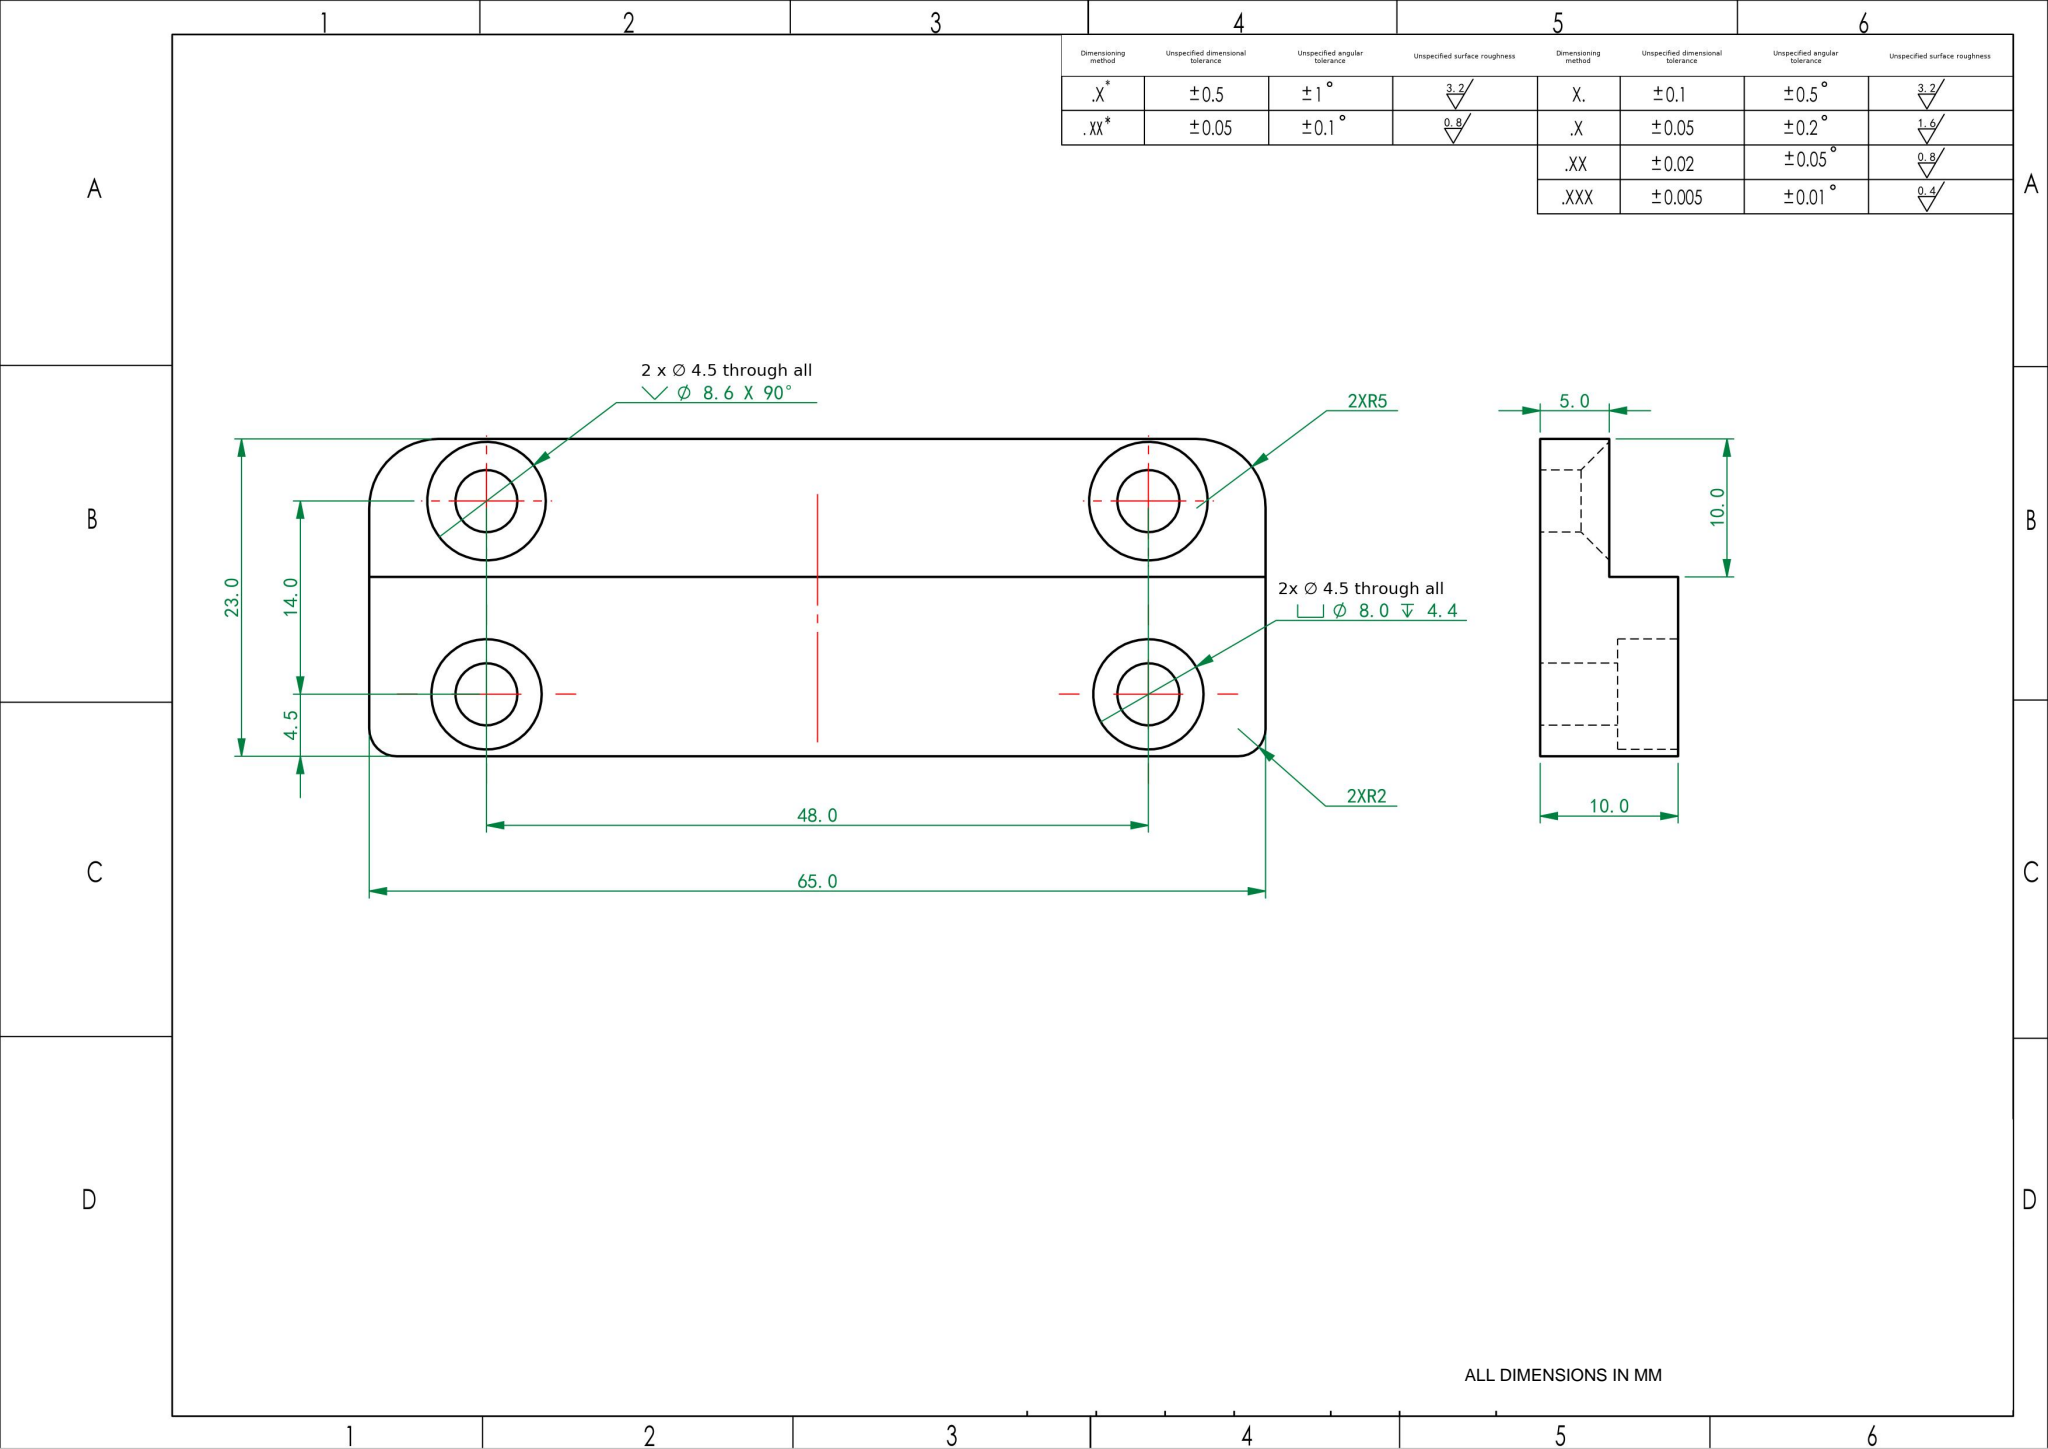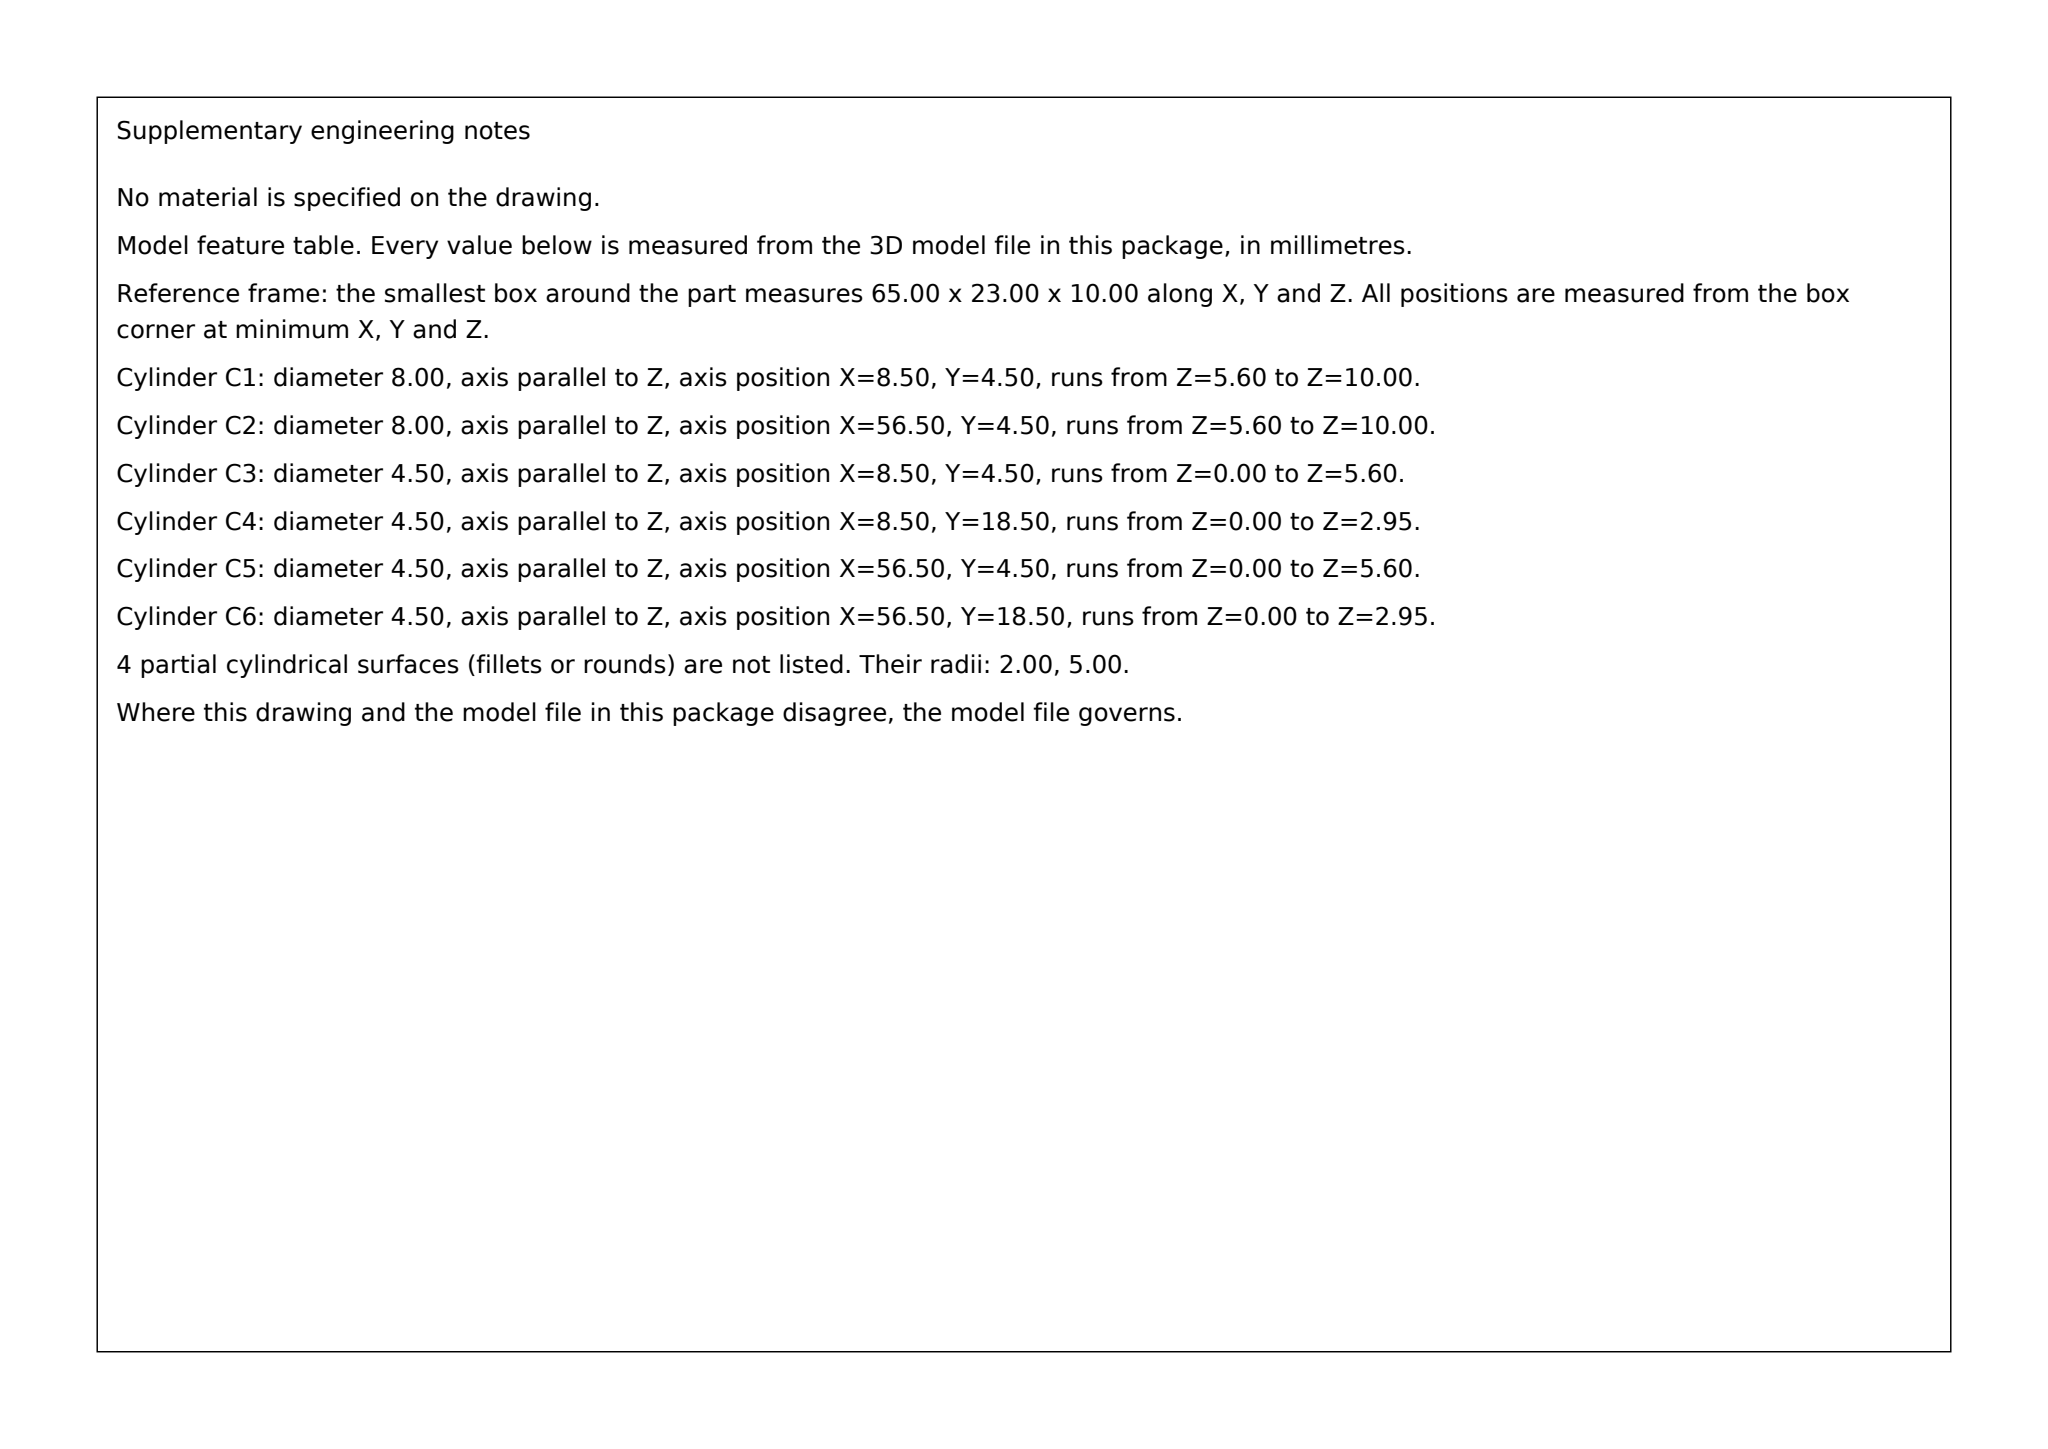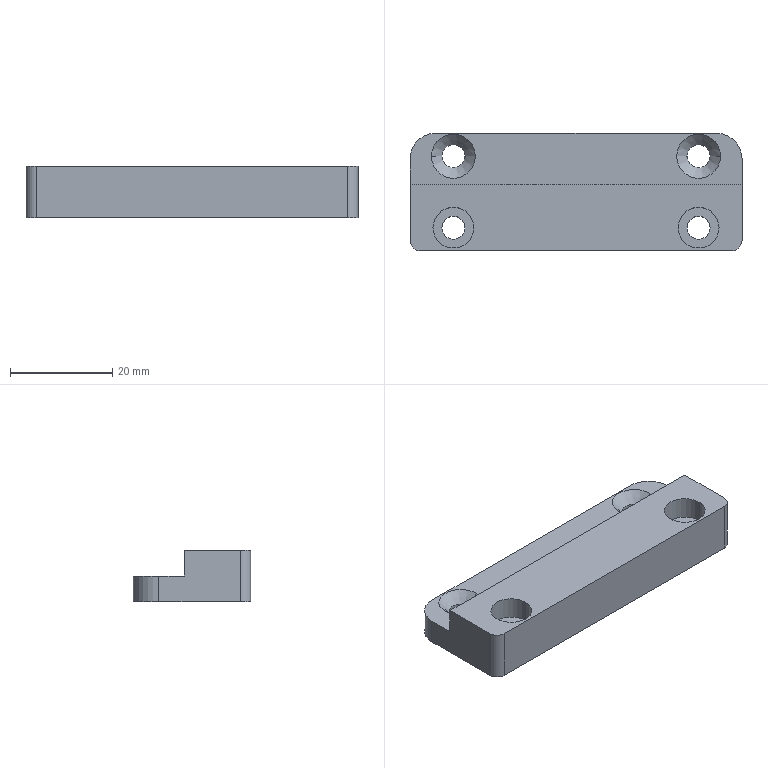Part | SolidWorks | mm | 1 solid | 30 faces | box 65 x 23 x 10 mm | volume 10772 mm3 | cylinder 16 | plane 10 | cone 4 | commonest cylinder face diameters 4.5 x8 8 x4 10 x2 4 x2
build123d program:
from build123d import *

# Parameters (mm, degrees)
SKETCH1_W                                         = 65
SKETCH1_H                                         = 23
BOSS_EXTRUDE1_DEPTH                               = 10
M4_HEX_SOCKET_HEAD_CAP_SCREW_CBORE2_D             = 4.5
M4_HEX_SOCKET_HEAD_CAP_SCREW_CBORE2_CBORE_D       = 8
M4_HEX_SOCKET_HEAD_CAP_SCREW_CBORE2_CBORE_DEPTH   = 4.4
SKETCH4_W                                         = 65
SKETCH4_H                                         = 10
CUT_EXTRUDE1_DEPTH                                = 5
FILLET1_R                                         = 5
FILLET2_R                                         = 2
HOLE_SIZE_ACCORDING_TO_PHILLIPS_COUNT_D           = 4.5
HOLE_SIZE_ACCORDING_TO_PHILLIPS_COUNT_CSINK_D     = 8.6
HOLE_SIZE_ACCORDING_TO_PHILLIPS_COUNT_CSINK_ANGLE = 90


with BuildPart() as part:
    # Sketch1 → Boss-Extrude1 (new body)
    with BuildSketch(Plane.XY):
        Rectangle(SKETCH1_W, SKETCH1_H)
    extrude(amount=BOSS_EXTRUDE1_DEPTH)

    # M4 Hex Socket Head Cap Screw CBORE2 (through all)
    with Locations(Plane(origin=(-24, 7, 10), x_dir=(1, 0, 0), z_dir=(0, 0, 1))):
        with Locations((0, 0), (0, -14), (48, -14), (48, 0)):
            CounterBoreHole(M4_HEX_SOCKET_HEAD_CAP_SCREW_CBORE2_D / 2, M4_HEX_SOCKET_HEAD_CAP_SCREW_CBORE2_CBORE_D / 2, M4_HEX_SOCKET_HEAD_CAP_SCREW_CBORE2_CBORE_DEPTH)

    # Sketch4 → Cut-Extrude1 (cut)
    with BuildSketch(Plane.XY.offset(10)):
        with Locations((0, 6.5)):
            Rectangle(SKETCH4_W, SKETCH4_H)
    extrude(amount=-CUT_EXTRUDE1_DEPTH, mode=Mode.SUBTRACT)

    # Fillet1
    fillet1_edges = [part.edges().sort_by_distance(p)[0] for p in [
        (-32.5, 11.5, 2.5),
        (32.5, 11.5, 2.5),
    ]]
    fillet(fillet1_edges, radius=FILLET1_R)

    # Fillet2
    fillet2_edges = [part.edges().sort_by_distance(p)[0] for p in [
        (32.5, -11.5, 5),
        (-32.5, -11.5, 5),
    ]]
    fillet(fillet2_edges, radius=FILLET2_R)

    # Hole Size _ according to Phillips_ Count (through all)
    with Locations(Plane(origin=(-24, 7, 5), x_dir=(1, 0, 0), z_dir=(0, 0, 1))):
        with Locations((0, 0), (48, 0)):
            CounterSinkHole(HOLE_SIZE_ACCORDING_TO_PHILLIPS_COUNT_D / 2, HOLE_SIZE_ACCORDING_TO_PHILLIPS_COUNT_CSINK_D / 2, counter_sink_angle=HOLE_SIZE_ACCORDING_TO_PHILLIPS_COUNT_CSINK_ANGLE)


solid = part.part